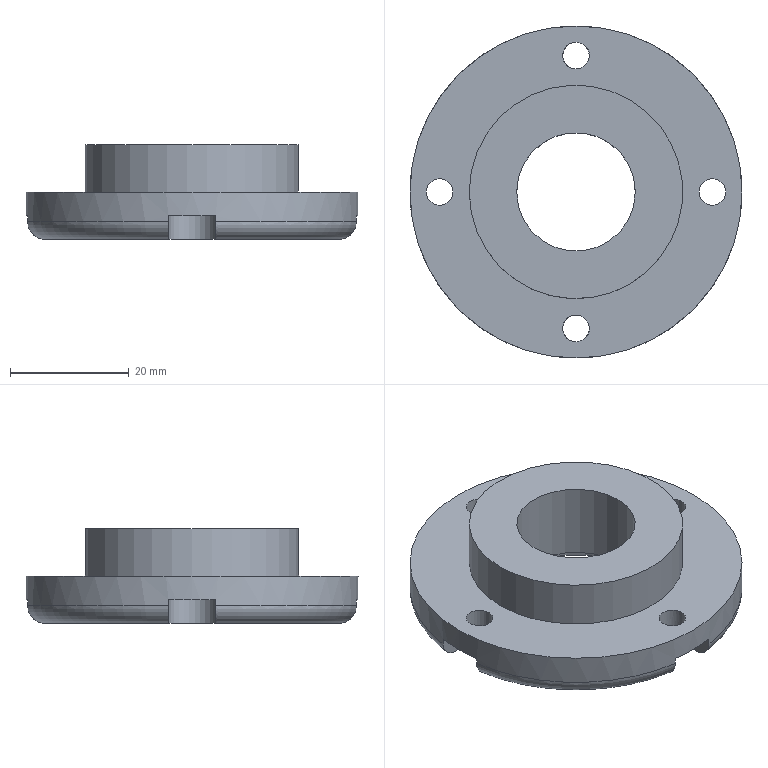Component | NX | 9 | 1 solid | 32 faces | volume 20491 mm3 | plane 16 | cylinder 12 | torus 4 | commonest cylinder face diameters 8 x4 4.5 x4 56 x1 36 x1 27 x1 20 x1